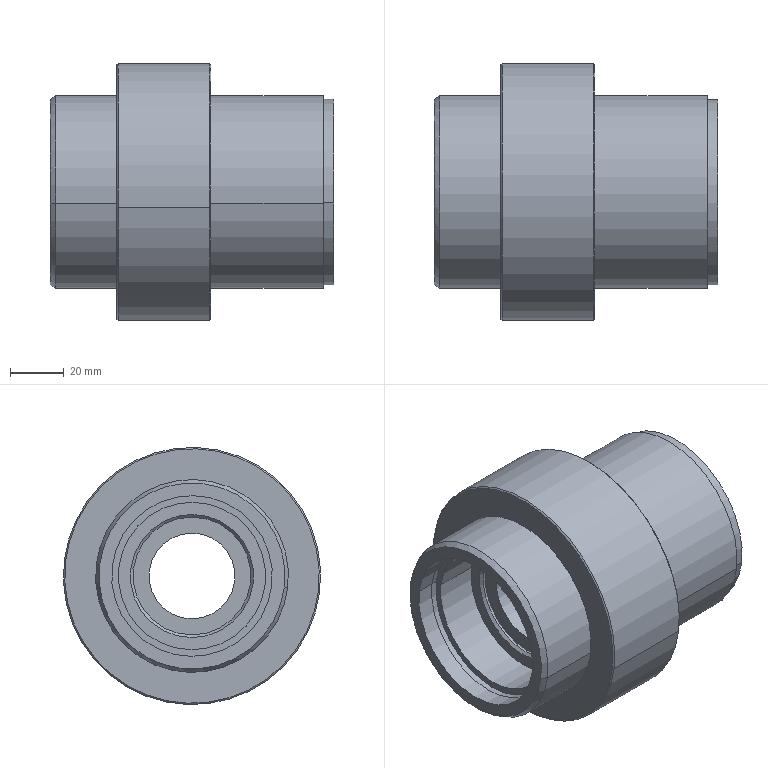Component | SolidWorks | 216InnerTubeAssembly-1_BearingSeat1-1 | 1 solid | 46 faces | box 106 x 96 x 96 mm | volume 363789 mm3 | cylinder 24 | plane 12 | cone 10 | commonest cylinder face diameters 72 x4 32 x4 60.01 x2 69.476 x2 56 x2 39 x2 44 x2 55 x2 | material Alloy Steel
build123d program:
from build123d import *

# Parameters (mm, degrees)
SKETCH1_W = 2.281
SKETCH1_H = 3.005


with BuildPart() as part:
    # Model → Revolve1 (revolve)
    with BuildSketch(Plane.XY, mode=Mode.PRIVATE) as revolve1_sk:
        Polygon((25, 23), (26, 22), (27, 22), (27, 16), (37, 16), (37, 19.5), (42.4, 19.5), (42.4, 16), (79, 16), (79, 28), (105, 28), (106, 29), (106, 34.738), (102, 34.738), (102, 36), (60, 36), (60, 47.5), (59.5, 48), (24.5, 48), (24, 47.5), (24, 36), (2.214, 36), (0, 34.722), (0, 30), (8, 30), (8, 27.5), (25, 27.5), (25, 27.361), align=None)
    revolve(revolve1_sk.sketch.rotate(Axis((-3.526, 0, 0), (1, 0, 0)), 180), axis=Axis((-3.526, 0, 0), (1, 0, 0)))

    # Sketch1 → Cut-Revolve1 (revolve, cut)
    with BuildSketch(Plane.XY, mode=Mode.PRIVATE) as cut_revolve1_sk:
        with Locations((7.863, 28.503)):
            Rectangle(SKETCH1_W, SKETCH1_H)
    revolve(cut_revolve1_sk.sketch.rotate(Axis((1.722, 0, 0), (1, 0, 0)), 180), axis=Axis((1.722, 0, 0), (1, 0, 0)), mode=Mode.SUBTRACT)

    # Sketch2 → Cut-Revolve2 (revolve, cut)
    with BuildSketch(Plane.XY, mode=Mode.PRIVATE) as cut_revolve2_sk:
        Polygon((23.522, 36), (25.006, 36), (25.006, 47.5), (25.506, 48), (25.506, 48.6), (23.522, 48.6), align=None)
    revolve(cut_revolve2_sk.sketch.rotate(Axis((18.522, 0, 0), (1, 0, 0)), 180), axis=Axis((18.522, 0, 0), (1, 0, 0)), mode=Mode.SUBTRACT)


solid = part.part

# Placed as in the assembly
solid = solid.moved(Location((895.278, 0, 0), (0, 0, 0)))